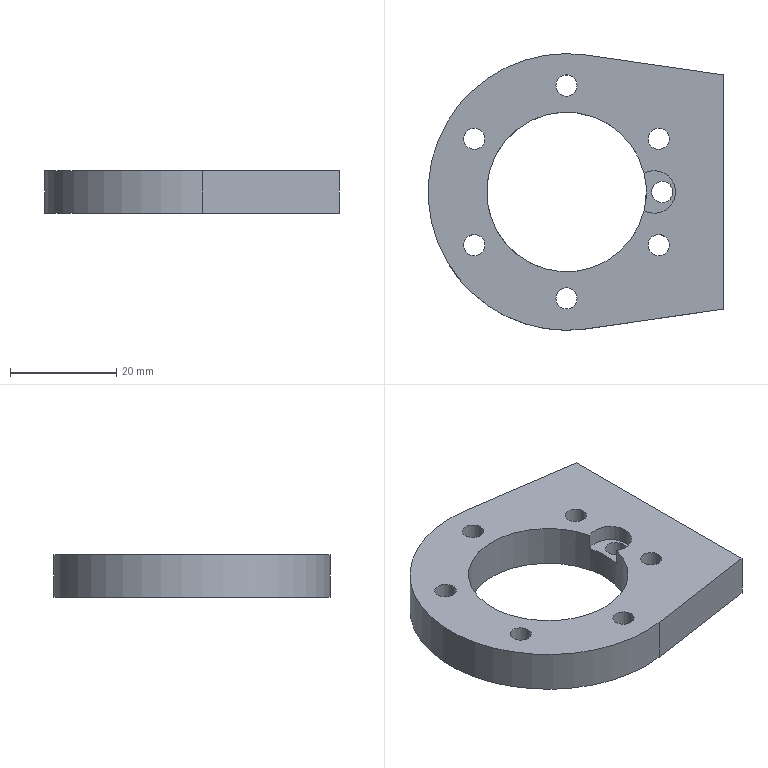Component | NX | 03B__27 | 1 solid | 20 faces | volume 13305 mm3 | cylinder 12 | plane 8 | commonest cylinder face diameters 4 x7 3 x2 52 x1 30 x1 8 x1